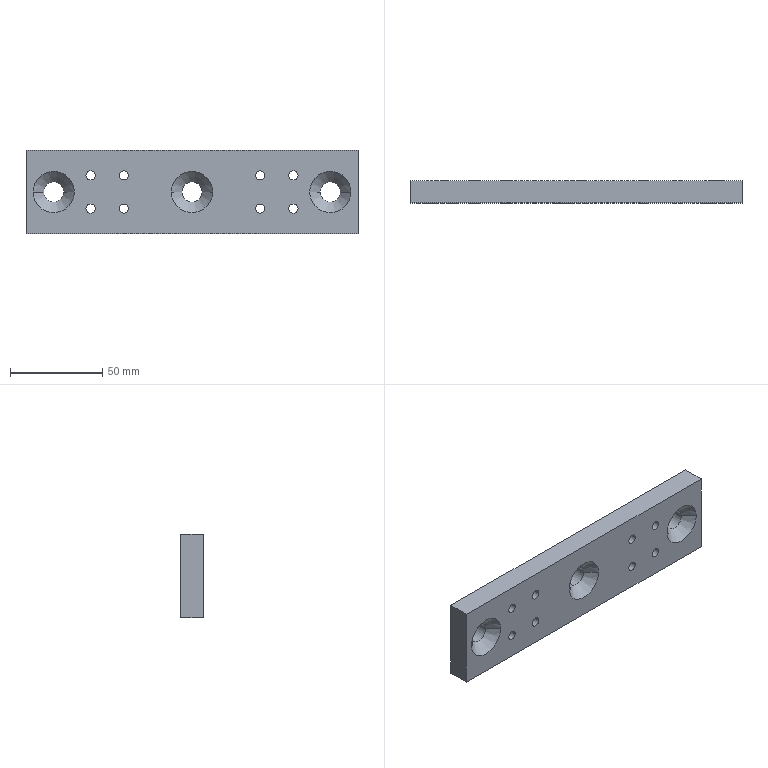Component | SolidWorks | YS01-054ClampingBlockMountingPlate-2 | 1 solid | 34 faces | box 180 x 12 x 45 mm | volume 89628 mm3 | cylinder 22 | cone 6 | plane 6 | commonest cylinder face diameters 5 x16 11 x6
STEP:
#1=COLOUR_RGB('',0.7922,0.8196,0.9333);
#2=FILL_AREA_STYLE_COLOUR('',#1);
#3=FILL_AREA_STYLE('',(#2));
#4=SURFACE_STYLE_FILL_AREA(#3);
#5=SURFACE_SIDE_STYLE('',(#4));
#6=SURFACE_STYLE_USAGE(.BOTH.,#5);
#7=PRESENTATION_STYLE_ASSIGNMENT((#6));
#8=CARTESIAN_POINT('',(-22.091,-12.408,94.425));
#9=VERTEX_POINT('',#8);
#10=CARTESIAN_POINT('',(-22.524,-12.408,94.425));
#11=VERTEX_POINT('',#10);
#12=CARTESIAN_POINT('',(-22.308,-12.408,94.425));
#13=DIRECTION('',(0.,-1.,0.));
#14=DIRECTION('',(-1.,0.,0.));
#15=AXIS2_PLACEMENT_3D('',#12,#13,#14);
#16=CIRCLE('',#15,0.2165);
#17=EDGE_CURVE('',#9,#11,#16,.T.);
#18=ORIENTED_EDGE('',*,*,#17,.F.);
#19=CARTESIAN_POINT('',(-21.867,-12.633,94.425));
#20=VERTEX_POINT('',#19);
#21=CARTESIAN_POINT('',(-21.867,-12.633,94.425));
#22=DIRECTION('',(0.7071,-0.7071,-0.));
#23=VECTOR('',#22,39.37);
#24=LINE('',#21,#23);
#25=EDGE_CURVE('',#9,#20,#24,.T.);
#26=ORIENTED_EDGE('',*,*,#25,.T.);
#27=CARTESIAN_POINT('',(-22.749,-12.633,94.425));
#28=VERTEX_POINT('',#27);
#29=CARTESIAN_POINT('',(-22.308,-12.633,94.425));
#30=DIRECTION('',(0.,-1.,0.));
#31=DIRECTION('',(-1.,0.,0.));
#32=AXIS2_PLACEMENT_3D('',#29,#30,#31);
#33=CIRCLE('',#32,0.4409);
#34=EDGE_CURVE('',#20,#28,#33,.T.);
#35=ORIENTED_EDGE('',*,*,#34,.T.);
#36=CARTESIAN_POINT('',(-22.749,-12.633,94.425));
#37=DIRECTION('',(-0.7071,-0.7071,0.));
#38=VECTOR('',#37,39.37);
#39=LINE('',#36,#38);
#40=EDGE_CURVE('',#11,#28,#39,.T.);
#41=ORIENTED_EDGE('',*,*,#40,.F.);
#42=EDGE_LOOP('',(#18,#26,#35,#41));
#43=FACE_OUTER_BOUND('',#42,.T.);
#44=CARTESIAN_POINT('',(-22.308,-12.633,94.425));
#45=DIRECTION('',(0.,-1.,0.));
#46=DIRECTION('',(-1.,0.,0.));
#47=AXIS2_PLACEMENT_3D('',#44,#45,#46);
#48=CONICAL_SURFACE('',#47,0.4409,0.7854);
#49=ADVANCED_FACE('',(#43),#48,.F.);
#50=CARTESIAN_POINT('',(-22.091,-12.16,94.425));
#51=VERTEX_POINT('',#50);
#52=CARTESIAN_POINT('',(-22.524,-12.16,94.425));
#53=VERTEX_POINT('',#52);
#54=CARTESIAN_POINT('',(-22.308,-12.16,94.425));
#55=DIRECTION('',(0.,-1.,0.));
#56=DIRECTION('',(-1.,0.,0.));
#57=AXIS2_PLACEMENT_3D('',#54,#55,#56);
#58=CIRCLE('',#57,0.2165);
#59=EDGE_CURVE('',#51,#53,#58,.T.);
#60=ORIENTED_EDGE('',*,*,#59,.F.);
#61=CARTESIAN_POINT('',(-22.091,-12.633,94.425));
#62=DIRECTION('',(0.,-1.,0.));
#63=VECTOR('',#62,39.37);
#64=LINE('',#61,#63);
#65=EDGE_CURVE('',#51,#9,#64,.T.);
#66=ORIENTED_EDGE('',*,*,#65,.T.);
#67=ORIENTED_EDGE('',*,*,#17,.T.);
#68=CARTESIAN_POINT('',(-22.524,-12.633,94.425));
#69=DIRECTION('',(0.,-1.,0.));
#70=VECTOR('',#69,39.37);
#71=LINE('',#68,#70);
#72=EDGE_CURVE('',#53,#11,#71,.T.);
#73=ORIENTED_EDGE('',*,*,#72,.F.);
#74=EDGE_LOOP('',(#60,#66,#67,#73));
#75=FACE_OUTER_BOUND('',#74,.T.);
#76=CARTESIAN_POINT('',(-22.308,-12.633,94.425));
#77=DIRECTION('',(0.,-1.,0.));
#78=DIRECTION('',(-1.,0.,0.));
#79=AXIS2_PLACEMENT_3D('',#76,#77,#78);
#80=CYLINDRICAL_SURFACE('',#79,0.2165);
#81=ADVANCED_FACE('',(#75),#80,.F.);
#82=CARTESIAN_POINT('',(-19.138,-12.408,94.425));
#83=VERTEX_POINT('',#82);
#84=CARTESIAN_POINT('',(-19.571,-12.408,94.425));
#85=VERTEX_POINT('',#84);
#86=CARTESIAN_POINT('',(-19.355,-12.408,94.425));
#87=DIRECTION('',(0.,-1.,0.));
#88=DIRECTION('',(-1.,0.,0.));
#89=AXIS2_PLACEMENT_3D('',#86,#87,#88);
#90=CIRCLE('',#89,0.2165);
#91=EDGE_CURVE('',#83,#85,#90,.T.);
#92=ORIENTED_EDGE('',*,*,#91,.F.);
#93=CARTESIAN_POINT('',(-18.914,-12.633,94.425));
#94=VERTEX_POINT('',#93);
#95=CARTESIAN_POINT('',(-18.914,-12.633,94.425));
#96=DIRECTION('',(0.7071,-0.7071,-0.));
#97=VECTOR('',#96,39.37);
#98=LINE('',#95,#97);
#99=EDGE_CURVE('',#83,#94,#98,.T.);
#100=ORIENTED_EDGE('',*,*,#99,.T.);
#101=CARTESIAN_POINT('',(-19.796,-12.633,94.425));
#102=VERTEX_POINT('',#101);
#103=CARTESIAN_POINT('',(-19.355,-12.633,94.425));
#104=DIRECTION('',(0.,-1.,0.));
#105=DIRECTION('',(-1.,0.,0.));
#106=AXIS2_PLACEMENT_3D('',#103,#104,#105);
#107=CIRCLE('',#106,0.4409);
#108=EDGE_CURVE('',#94,#102,#107,.T.);
#109=ORIENTED_EDGE('',*,*,#108,.T.);
#110=CARTESIAN_POINT('',(-19.796,-12.633,94.425));
#111=DIRECTION('',(-0.7071,-0.7071,0.));
#112=VECTOR('',#111,39.37);
#113=LINE('',#110,#112);
#114=EDGE_CURVE('',#85,#102,#113,.T.);
#115=ORIENTED_EDGE('',*,*,#114,.F.);
#116=EDGE_LOOP('',(#92,#100,#109,#115));
#117=FACE_OUTER_BOUND('',#116,.T.);
#118=CARTESIAN_POINT('',(-19.355,-12.633,94.425));
#119=DIRECTION('',(0.,-1.,0.));
#120=DIRECTION('',(-1.,0.,0.));
#121=AXIS2_PLACEMENT_3D('',#118,#119,#120);
#122=CONICAL_SURFACE('',#121,0.4409,0.7854);
#123=ADVANCED_FACE('',(#117),#122,.F.);
#124=CARTESIAN_POINT('',(-19.138,-12.16,94.425));
#125=VERTEX_POINT('',#124);
#126=CARTESIAN_POINT('',(-19.571,-12.16,94.425));
#127=VERTEX_POINT('',#126);
#128=CARTESIAN_POINT('',(-19.355,-12.16,94.425));
#129=DIRECTION('',(0.,-1.,0.));
#130=DIRECTION('',(-1.,0.,0.));
#131=AXIS2_PLACEMENT_3D('',#128,#129,#130);
#132=CIRCLE('',#131,0.2165);
#133=EDGE_CURVE('',#125,#127,#132,.T.);
#134=ORIENTED_EDGE('',*,*,#133,.F.);
#135=CARTESIAN_POINT('',(-19.138,-12.633,94.425));
#136=DIRECTION('',(0.,-1.,0.));
#137=VECTOR('',#136,39.37);
#138=LINE('',#135,#137);
#139=EDGE_CURVE('',#125,#83,#138,.T.);
#140=ORIENTED_EDGE('',*,*,#139,.T.);
#141=ORIENTED_EDGE('',*,*,#91,.T.);
#142=CARTESIAN_POINT('',(-19.571,-12.633,94.425));
#143=DIRECTION('',(0.,-1.,0.));
#144=VECTOR('',#143,39.37);
#145=LINE('',#142,#144);
#146=EDGE_CURVE('',#127,#85,#145,.T.);
#147=ORIENTED_EDGE('',*,*,#146,.F.);
#148=EDGE_LOOP('',(#134,#140,#141,#147));
#149=FACE_OUTER_BOUND('',#148,.T.);
#150=CARTESIAN_POINT('',(-19.355,-12.633,94.425));
#151=DIRECTION('',(0.,-1.,0.));
#152=DIRECTION('',(-1.,0.,0.));
#153=AXIS2_PLACEMENT_3D('',#150,#151,#152);
#154=CYLINDRICAL_SURFACE('',#153,0.2165);
#155=ADVANCED_FACE('',(#149),#154,.F.);
#156=CARTESIAN_POINT('',(-25.044,-12.408,94.425));
#157=VERTEX_POINT('',#156);
#158=CARTESIAN_POINT('',(-25.477,-12.408,94.425));
#159=VERTEX_POINT('',#158);
#160=CARTESIAN_POINT('',(-25.26,-12.408,94.425));
#161=DIRECTION('',(0.,-1.,0.));
#162=DIRECTION('',(-1.,0.,0.));
#163=AXIS2_PLACEMENT_3D('',#160,#161,#162);
#164=CIRCLE('',#163,0.2165);
#165=EDGE_CURVE('',#157,#159,#164,.T.);
#166=ORIENTED_EDGE('',*,*,#165,.F.);
#167=CARTESIAN_POINT('',(-24.819,-12.633,94.425));
#168=VERTEX_POINT('',#167);
#169=CARTESIAN_POINT('',(-24.819,-12.633,94.425));
#170=DIRECTION('',(0.7071,-0.7071,-0.));
#171=VECTOR('',#170,39.37);
#172=LINE('',#169,#171);
#173=EDGE_CURVE('',#157,#168,#172,.T.);
#174=ORIENTED_EDGE('',*,*,#173,.T.);
#175=CARTESIAN_POINT('',(-25.701,-12.633,94.425));
#176=VERTEX_POINT('',#175);
#177=CARTESIAN_POINT('',(-25.26,-12.633,94.425));
#178=DIRECTION('',(0.,-1.,0.));
#179=DIRECTION('',(-1.,0.,0.));
#180=AXIS2_PLACEMENT_3D('',#177,#178,#179);
#181=CIRCLE('',#180,0.4409);
#182=EDGE_CURVE('',#168,#176,#181,.T.);
#183=ORIENTED_EDGE('',*,*,#182,.T.);
#184=CARTESIAN_POINT('',(-25.701,-12.633,94.425));
#185=DIRECTION('',(-0.7071,-0.7071,0.));
#186=VECTOR('',#185,39.37);
#187=LINE('',#184,#186);
#188=EDGE_CURVE('',#159,#176,#187,.T.);
#189=ORIENTED_EDGE('',*,*,#188,.F.);
#190=EDGE_LOOP('',(#166,#174,#183,#189));
#191=FACE_OUTER_BOUND('',#190,.T.);
#192=CARTESIAN_POINT('',(-25.26,-12.633,94.425));
#193=DIRECTION('',(0.,-1.,0.));
#194=DIRECTION('',(-1.,0.,0.));
#195=AXIS2_PLACEMENT_3D('',#192,#193,#194);
#196=CONICAL_SURFACE('',#195,0.4409,0.7854);
#197=ADVANCED_FACE('',(#191),#196,.F.);
#198=CARTESIAN_POINT('',(-25.044,-12.16,94.425));
#199=VERTEX_POINT('',#198);
#200=CARTESIAN_POINT('',(-25.477,-12.16,94.425));
#201=VERTEX_POINT('',#200);
#202=CARTESIAN_POINT('',(-25.26,-12.16,94.425));
#203=DIRECTION('',(0.,-1.,0.));
#204=DIRECTION('',(-1.,0.,0.));
#205=AXIS2_PLACEMENT_3D('',#202,#203,#204);
#206=CIRCLE('',#205,0.2165);
#207=EDGE_CURVE('',#199,#201,#206,.T.);
#208=ORIENTED_EDGE('',*,*,#207,.F.);
#209=CARTESIAN_POINT('',(-25.044,-12.633,94.425));
#210=DIRECTION('',(0.,-1.,0.));
#211=VECTOR('',#210,39.37);
#212=LINE('',#209,#211);
#213=EDGE_CURVE('',#199,#157,#212,.T.);
#214=ORIENTED_EDGE('',*,*,#213,.T.);
#215=ORIENTED_EDGE('',*,*,#165,.T.);
#216=CARTESIAN_POINT('',(-25.477,-12.633,94.425));
#217=DIRECTION('',(0.,-1.,0.));
#218=VECTOR('',#217,39.37);
#219=LINE('',#216,#218);
#220=EDGE_CURVE('',#201,#159,#219,.T.);
#221=ORIENTED_EDGE('',*,*,#220,.F.);
#222=EDGE_LOOP('',(#208,#214,#215,#221));
#223=FACE_OUTER_BOUND('',#222,.T.);
#224=CARTESIAN_POINT('',(-25.26,-12.633,94.425));
#225=DIRECTION('',(0.,-1.,0.));
#226=DIRECTION('',(-1.,0.,0.));
#227=AXIS2_PLACEMENT_3D('',#224,#225,#226);
#228=CYLINDRICAL_SURFACE('',#227,0.2165);
#229=ADVANCED_FACE('',(#223),#228,.F.);
#230=CARTESIAN_POINT('',(-23.863,-12.16,94.071));
#231=VERTEX_POINT('',#230);
#232=CARTESIAN_POINT('',(-23.666,-12.16,94.071));
#233=VERTEX_POINT('',#232);
#234=CARTESIAN_POINT('',(-23.764,-12.16,94.071));
#235=DIRECTION('',(-0.,1.,0.));
#236=DIRECTION('',(1.,0.,0.));
#237=AXIS2_PLACEMENT_3D('',#234,#235,#236);
#238=CIRCLE('',#237,0.09843);
#239=EDGE_CURVE('',#231,#233,#238,.T.);
#240=ORIENTED_EDGE('',*,*,#239,.T.);
#241=CARTESIAN_POINT('',(-23.666,-12.633,94.071));
#242=VERTEX_POINT('',#241);
#243=CARTESIAN_POINT('',(-23.666,-12.633,94.071));
#244=DIRECTION('',(0.,-1.,0.));
#245=VECTOR('',#244,39.37);
#246=LINE('',#243,#245);
#247=EDGE_CURVE('',#233,#242,#246,.T.);
#248=ORIENTED_EDGE('',*,*,#247,.T.);
#249=CARTESIAN_POINT('',(-23.863,-12.633,94.071));
#250=VERTEX_POINT('',#249);
#251=CARTESIAN_POINT('',(-23.764,-12.633,94.071));
#252=DIRECTION('',(0.,-1.,0.));
#253=DIRECTION('',(-1.,0.,0.));
#254=AXIS2_PLACEMENT_3D('',#251,#252,#253);
#255=CIRCLE('',#254,0.09843);
#256=EDGE_CURVE('',#242,#250,#255,.T.);
#257=ORIENTED_EDGE('',*,*,#256,.T.);
#258=CARTESIAN_POINT('',(-23.863,-12.633,94.071));
#259=DIRECTION('',(0.,-1.,0.));
#260=VECTOR('',#259,39.37);
#261=LINE('',#258,#260);
#262=EDGE_CURVE('',#231,#250,#261,.T.);
#263=ORIENTED_EDGE('',*,*,#262,.F.);
#264=EDGE_LOOP('',(#240,#248,#257,#263));
#265=FACE_OUTER_BOUND('',#264,.T.);
#266=CARTESIAN_POINT('',(-23.764,-12.633,94.071));
#267=DIRECTION('',(0.,-1.,0.));
#268=DIRECTION('',(-1.,0.,0.));
#269=AXIS2_PLACEMENT_3D('',#266,#267,#268);
#270=CYLINDRICAL_SURFACE('',#269,0.09843);
#271=ADVANCED_FACE('',(#265),#270,.F.);
#272=CARTESIAN_POINT('',(-20.949,-12.16,94.071));
#273=VERTEX_POINT('',#272);
#274=CARTESIAN_POINT('',(-20.752,-12.16,94.071));
#275=VERTEX_POINT('',#274);
#276=CARTESIAN_POINT('',(-20.851,-12.16,94.071));
#277=DIRECTION('',(-0.,1.,0.));
#278=DIRECTION('',(1.,0.,0.));
#279=AXIS2_PLACEMENT_3D('',#276,#277,#278);
#280=CIRCLE('',#279,0.09843);
#281=EDGE_CURVE('',#273,#275,#280,.T.);
#282=ORIENTED_EDGE('',*,*,#281,.T.);
#283=CARTESIAN_POINT('',(-20.752,-12.633,94.071));
#284=VERTEX_POINT('',#283);
#285=CARTESIAN_POINT('',(-20.752,-12.633,94.071));
#286=DIRECTION('',(0.,-1.,0.));
#287=VECTOR('',#286,39.37);
#288=LINE('',#285,#287);
#289=EDGE_CURVE('',#275,#284,#288,.T.);
#290=ORIENTED_EDGE('',*,*,#289,.T.);
#291=CARTESIAN_POINT('',(-20.949,-12.633,94.071));
#292=VERTEX_POINT('',#291);
#293=CARTESIAN_POINT('',(-20.851,-12.633,94.071));
#294=DIRECTION('',(0.,-1.,0.));
#295=DIRECTION('',(-1.,0.,0.));
#296=AXIS2_PLACEMENT_3D('',#293,#294,#295);
#297=CIRCLE('',#296,0.09843);
#298=EDGE_CURVE('',#284,#292,#297,.T.);
#299=ORIENTED_EDGE('',*,*,#298,.T.);
#300=CARTESIAN_POINT('',(-20.949,-12.633,94.071));
#301=DIRECTION('',(0.,-1.,0.));
#302=VECTOR('',#301,39.37);
#303=LINE('',#300,#302);
#304=EDGE_CURVE('',#273,#292,#303,.T.);
#305=ORIENTED_EDGE('',*,*,#304,.F.);
#306=EDGE_LOOP('',(#282,#290,#299,#305));
#307=FACE_OUTER_BOUND('',#306,.T.);
#308=CARTESIAN_POINT('',(-20.851,-12.633,94.071));
#309=DIRECTION('',(0.,-1.,0.));
#310=DIRECTION('',(-1.,0.,0.));
#311=AXIS2_PLACEMENT_3D('',#308,#309,#310);
#312=CYLINDRICAL_SURFACE('',#311,0.09843);
#313=ADVANCED_FACE('',(#307),#312,.F.);
#314=CARTESIAN_POINT('',(-23.863,-12.16,94.78));
#315=VERTEX_POINT('',#314);
#316=CARTESIAN_POINT('',(-23.666,-12.16,94.78));
#317=VERTEX_POINT('',#316);
#318=CARTESIAN_POINT('',(-23.764,-12.16,94.78));
#319=DIRECTION('',(-0.,1.,0.));
#320=DIRECTION('',(1.,0.,0.));
#321=AXIS2_PLACEMENT_3D('',#318,#319,#320);
#322=CIRCLE('',#321,0.09843);
#323=EDGE_CURVE('',#315,#317,#322,.T.);
#324=ORIENTED_EDGE('',*,*,#323,.T.);
#325=CARTESIAN_POINT('',(-23.666,-12.633,94.78));
#326=VERTEX_POINT('',#325);
#327=CARTESIAN_POINT('',(-23.666,-12.633,94.78));
#328=DIRECTION('',(0.,-1.,0.));
#329=VECTOR('',#328,39.37);
#330=LINE('',#327,#329);
#331=EDGE_CURVE('',#317,#326,#330,.T.);
#332=ORIENTED_EDGE('',*,*,#331,.T.);
#333=CARTESIAN_POINT('',(-23.863,-12.633,94.78));
#334=VERTEX_POINT('',#333);
#335=CARTESIAN_POINT('',(-23.764,-12.633,94.78));
#336=DIRECTION('',(0.,-1.,0.));
#337=DIRECTION('',(-1.,0.,0.));
#338=AXIS2_PLACEMENT_3D('',#335,#336,#337);
#339=CIRCLE('',#338,0.09843);
#340=EDGE_CURVE('',#326,#334,#339,.T.);
#341=ORIENTED_EDGE('',*,*,#340,.T.);
#342=CARTESIAN_POINT('',(-23.863,-12.633,94.78));
#343=DIRECTION('',(0.,-1.,0.));
#344=VECTOR('',#343,39.37);
#345=LINE('',#342,#344);
#346=EDGE_CURVE('',#315,#334,#345,.T.);
#347=ORIENTED_EDGE('',*,*,#346,.F.);
#348=EDGE_LOOP('',(#324,#332,#341,#347));
#349=FACE_OUTER_BOUND('',#348,.T.);
#350=CARTESIAN_POINT('',(-23.764,-12.633,94.78));
#351=DIRECTION('',(0.,-1.,0.));
#352=DIRECTION('',(-1.,0.,0.));
#353=AXIS2_PLACEMENT_3D('',#350,#351,#352);
#354=CYLINDRICAL_SURFACE('',#353,0.09843);
#355=ADVANCED_FACE('',(#349),#354,.F.);
#356=CARTESIAN_POINT('',(-20.949,-12.16,94.78));
#357=VERTEX_POINT('',#356);
#358=CARTESIAN_POINT('',(-20.752,-12.16,94.78));
#359=VERTEX_POINT('',#358);
#360=CARTESIAN_POINT('',(-20.851,-12.16,94.78));
#361=DIRECTION('',(-0.,1.,0.));
#362=DIRECTION('',(1.,0.,0.));
#363=AXIS2_PLACEMENT_3D('',#360,#361,#362);
#364=CIRCLE('',#363,0.09843);
#365=EDGE_CURVE('',#357,#359,#364,.T.);
#366=ORIENTED_EDGE('',*,*,#365,.T.);
#367=CARTESIAN_POINT('',(-20.752,-12.633,94.78));
#368=VERTEX_POINT('',#367);
#369=CARTESIAN_POINT('',(-20.752,-12.633,94.78));
#370=DIRECTION('',(0.,-1.,0.));
#371=VECTOR('',#370,39.37);
#372=LINE('',#369,#371);
#373=EDGE_CURVE('',#359,#368,#372,.T.);
#374=ORIENTED_EDGE('',*,*,#373,.T.);
#375=CARTESIAN_POINT('',(-20.949,-12.633,94.78));
#376=VERTEX_POINT('',#375);
#377=CARTESIAN_POINT('',(-20.851,-12.633,94.78));
#378=DIRECTION('',(0.,-1.,0.));
#379=DIRECTION('',(-1.,0.,0.));
#380=AXIS2_PLACEMENT_3D('',#377,#378,#379);
#381=CIRCLE('',#380,0.09843);
#382=EDGE_CURVE('',#368,#376,#381,.T.);
#383=ORIENTED_EDGE('',*,*,#382,.T.);
#384=CARTESIAN_POINT('',(-20.949,-12.633,94.78));
#385=DIRECTION('',(0.,-1.,0.));
#386=VECTOR('',#385,39.37);
#387=LINE('',#384,#386);
#388=EDGE_CURVE('',#357,#376,#387,.T.);
#389=ORIENTED_EDGE('',*,*,#388,.F.);
#390=EDGE_LOOP('',(#366,#374,#383,#389));
#391=FACE_OUTER_BOUND('',#390,.T.);
#392=CARTESIAN_POINT('',(-20.851,-12.633,94.78));
#393=DIRECTION('',(0.,-1.,0.));
#394=DIRECTION('',(-1.,0.,0.));
#395=AXIS2_PLACEMENT_3D('',#392,#393,#394);
#396=CYLINDRICAL_SURFACE('',#395,0.09843);
#397=ADVANCED_FACE('',(#391),#396,.F.);
#398=CARTESIAN_POINT('',(-24.571,-12.16,94.78));
#399=VERTEX_POINT('',#398);
#400=CARTESIAN_POINT('',(-24.374,-12.16,94.78));
#401=VERTEX_POINT('',#400);
#402=CARTESIAN_POINT('',(-24.473,-12.16,94.78));
#403=DIRECTION('',(-0.,1.,0.));
#404=DIRECTION('',(1.,0.,0.));
#405=AXIS2_PLACEMENT_3D('',#402,#403,#404);
#406=CIRCLE('',#405,0.09843);
#407=EDGE_CURVE('',#399,#401,#406,.T.);
#408=ORIENTED_EDGE('',*,*,#407,.T.);
#409=CARTESIAN_POINT('',(-24.374,-12.633,94.78));
#410=VERTEX_POINT('',#409);
#411=CARTESIAN_POINT('',(-24.374,-12.633,94.78));
#412=DIRECTION('',(0.,-1.,0.));
#413=VECTOR('',#412,39.37);
#414=LINE('',#411,#413);
#415=EDGE_CURVE('',#401,#410,#414,.T.);
#416=ORIENTED_EDGE('',*,*,#415,.T.);
#417=CARTESIAN_POINT('',(-24.571,-12.633,94.78));
#418=VERTEX_POINT('',#417);
#419=CARTESIAN_POINT('',(-24.473,-12.633,94.78));
#420=DIRECTION('',(0.,-1.,0.));
#421=DIRECTION('',(-1.,0.,0.));
#422=AXIS2_PLACEMENT_3D('',#419,#420,#421);
#423=CIRCLE('',#422,0.09843);
#424=EDGE_CURVE('',#410,#418,#423,.T.);
#425=ORIENTED_EDGE('',*,*,#424,.T.);
#426=CARTESIAN_POINT('',(-24.571,-12.633,94.78));
#427=DIRECTION('',(0.,-1.,0.));
#428=VECTOR('',#427,39.37);
#429=LINE('',#426,#428);
#430=EDGE_CURVE('',#399,#418,#429,.T.);
#431=ORIENTED_EDGE('',*,*,#430,.F.);
#432=EDGE_LOOP('',(#408,#416,#425,#431));
#433=FACE_OUTER_BOUND('',#432,.T.);
#434=CARTESIAN_POINT('',(-24.473,-12.633,94.78));
#435=DIRECTION('',(0.,-1.,0.));
#436=DIRECTION('',(-1.,0.,0.));
#437=AXIS2_PLACEMENT_3D('',#434,#435,#436);
#438=CYLINDRICAL_SURFACE('',#437,0.09843);
#439=ADVANCED_FACE('',(#433),#438,.F.);
#440=CARTESIAN_POINT('',(-24.571,-12.16,94.071));
#441=VERTEX_POINT('',#440);
#442=CARTESIAN_POINT('',(-24.374,-12.16,94.071));
#443=VERTEX_POINT('',#442);
#444=CARTESIAN_POINT('',(-24.473,-12.16,94.071));
#445=DIRECTION('',(-0.,1.,0.));
#446=DIRECTION('',(1.,0.,0.));
#447=AXIS2_PLACEMENT_3D('',#444,#445,#446);
#448=CIRCLE('',#447,0.09843);
#449=EDGE_CURVE('',#441,#443,#448,.T.);
#450=ORIENTED_EDGE('',*,*,#449,.T.);
#451=CARTESIAN_POINT('',(-24.374,-12.633,94.071));
#452=VERTEX_POINT('',#451);
#453=CARTESIAN_POINT('',(-24.374,-12.633,94.071));
#454=DIRECTION('',(0.,-1.,0.));
#455=VECTOR('',#454,39.37);
#456=LINE('',#453,#455);
#457=EDGE_CURVE('',#443,#452,#456,.T.);
#458=ORIENTED_EDGE('',*,*,#457,.T.);
#459=CARTESIAN_POINT('',(-24.571,-12.633,94.071));
#460=VERTEX_POINT('',#459);
#461=CARTESIAN_POINT('',(-24.473,-12.633,94.071));
#462=DIRECTION('',(0.,-1.,0.));
#463=DIRECTION('',(-1.,0.,0.));
#464=AXIS2_PLACEMENT_3D('',#461,#462,#463);
#465=CIRCLE('',#464,0.09843);
#466=EDGE_CURVE('',#452,#460,#465,.T.);
#467=ORIENTED_EDGE('',*,*,#466,.T.);
#468=CARTESIAN_POINT('',(-24.571,-12.633,94.071));
#469=DIRECTION('',(0.,-1.,0.));
#470=VECTOR('',#469,39.37);
#471=LINE('',#468,#470);
#472=EDGE_CURVE('',#441,#460,#471,.T.);
#473=ORIENTED_EDGE('',*,*,#472,.F.);
#474=EDGE_LOOP('',(#450,#458,#467,#473));
#475=FACE_OUTER_BOUND('',#474,.T.);
#476=CARTESIAN_POINT('',(-24.473,-12.633,94.071));
#477=DIRECTION('',(0.,-1.,0.));
#478=DIRECTION('',(-1.,0.,0.));
#479=AXIS2_PLACEMENT_3D('',#476,#477,#478);
#480=CYLINDRICAL_SURFACE('',#479,0.09843);
#481=ADVANCED_FACE('',(#475),#480,.F.);
#482=CARTESIAN_POINT('',(-20.241,-12.16,94.78));
#483=VERTEX_POINT('',#482);
#484=CARTESIAN_POINT('',(-20.044,-12.16,94.78));
#485=VERTEX_POINT('',#484);
#486=CARTESIAN_POINT('',(-20.142,-12.16,94.78));
#487=DIRECTION('',(-0.,1.,0.));
#488=DIRECTION('',(1.,0.,0.));
#489=AXIS2_PLACEMENT_3D('',#486,#487,#488);
#490=CIRCLE('',#489,0.09843);
#491=EDGE_CURVE('',#483,#485,#490,.T.);
#492=ORIENTED_EDGE('',*,*,#491,.T.);
#493=CARTESIAN_POINT('',(-20.044,-12.633,94.78));
#494=VERTEX_POINT('',#493);
#495=CARTESIAN_POINT('',(-20.044,-12.633,94.78));
#496=DIRECTION('',(0.,-1.,0.));
#497=VECTOR('',#496,39.37);
#498=LINE('',#495,#497);
#499=EDGE_CURVE('',#485,#494,#498,.T.);
#500=ORIENTED_EDGE('',*,*,#499,.T.);
#501=CARTESIAN_POINT('',(-20.241,-12.633,94.78));
#502=VERTEX_POINT('',#501);
#503=CARTESIAN_POINT('',(-20.142,-12.633,94.78));
#504=DIRECTION('',(0.,-1.,0.));
#505=DIRECTION('',(-1.,0.,0.));
#506=AXIS2_PLACEMENT_3D('',#503,#504,#505);
#507=CIRCLE('',#506,0.09843);
#508=EDGE_CURVE('',#494,#502,#507,.T.);
#509=ORIENTED_EDGE('',*,*,#508,.T.);
#510=CARTESIAN_POINT('',(-20.241,-12.633,94.78));
#511=DIRECTION('',(0.,-1.,0.));
#512=VECTOR('',#511,39.37);
#513=LINE('',#510,#512);
#514=EDGE_CURVE('',#483,#502,#513,.T.);
#515=ORIENTED_EDGE('',*,*,#514,.F.);
#516=EDGE_LOOP('',(#492,#500,#509,#515));
#517=FACE_OUTER_BOUND('',#516,.T.);
#518=CARTESIAN_POINT('',(-20.142,-12.633,94.78));
#519=DIRECTION('',(0.,-1.,0.));
#520=DIRECTION('',(-1.,0.,0.));
#521=AXIS2_PLACEMENT_3D('',#518,#519,#520);
#522=CYLINDRICAL_SURFACE('',#521,0.09843);
#523=ADVANCED_FACE('',(#517),#522,.F.);
#524=CARTESIAN_POINT('',(-20.241,-12.16,94.071));
#525=VERTEX_POINT('',#524);
#526=CARTESIAN_POINT('',(-20.044,-12.16,94.071));
#527=VERTEX_POINT('',#526);
#528=CARTESIAN_POINT('',(-20.142,-12.16,94.071));
#529=DIRECTION('',(-0.,1.,0.));
#530=DIRECTION('',(1.,0.,0.));
#531=AXIS2_PLACEMENT_3D('',#528,#529,#530);
#532=CIRCLE('',#531,0.09843);
#533=EDGE_CURVE('',#525,#527,#532,.T.);
#534=ORIENTED_EDGE('',*,*,#533,.T.);
#535=CARTESIAN_POINT('',(-20.044,-12.633,94.071));
#536=VERTEX_POINT('',#535);
#537=CARTESIAN_POINT('',(-20.044,-12.633,94.071));
#538=DIRECTION('',(0.,-1.,0.));
#539=VECTOR('',#538,39.37);
#540=LINE('',#537,#539);
#541=EDGE_CURVE('',#527,#536,#540,.T.);
#542=ORIENTED_EDGE('',*,*,#541,.T.);
#543=CARTESIAN_POINT('',(-20.241,-12.633,94.071));
#544=VERTEX_POINT('',#543);
#545=CARTESIAN_POINT('',(-20.142,-12.633,94.071));
#546=DIRECTION('',(0.,-1.,0.));
#547=DIRECTION('',(-1.,0.,0.));
#548=AXIS2_PLACEMENT_3D('',#545,#546,#547);
#549=CIRCLE('',#548,0.09843);
#550=EDGE_CURVE('',#536,#544,#549,.T.);
#551=ORIENTED_EDGE('',*,*,#550,.T.);
#552=CARTESIAN_POINT('',(-20.241,-12.633,94.071));
#553=DIRECTION('',(0.,-1.,0.));
#554=VECTOR('',#553,39.37);
#555=LINE('',#552,#554);
#556=EDGE_CURVE('',#525,#544,#555,.T.);
#557=ORIENTED_EDGE('',*,*,#556,.F.);
#558=EDGE_LOOP('',(#534,#542,#551,#557));
#559=FACE_OUTER_BOUND('',#558,.T.);
#560=CARTESIAN_POINT('',(-20.142,-12.633,94.071));
#561=DIRECTION('',(0.,-1.,0.));
#562=DIRECTION('',(-1.,0.,0.));
#563=AXIS2_PLACEMENT_3D('',#560,#561,#562);
#564=CYLINDRICAL_SURFACE('',#563,0.09843);
#565=ADVANCED_FACE('',(#559),#564,.F.);
#566=CARTESIAN_POINT('',(-22.308,-12.633,94.425));
#567=DIRECTION('',(0.,-1.,0.));
#568=DIRECTION('',(-1.,0.,0.));
#569=AXIS2_PLACEMENT_3D('',#566,#567,#568);
#570=CIRCLE('',#569,0.4409);
#571=EDGE_CURVE('',#28,#20,#570,.T.);
#572=ORIENTED_EDGE('',*,*,#571,.F.);
#573=ORIENTED_EDGE('',*,*,#34,.F.);
#574=EDGE_LOOP('',(#572,#573));
#575=FACE_BOUND('',#574,.T.);
#576=CARTESIAN_POINT('',(-19.355,-12.633,94.425));
#577=DIRECTION('',(0.,-1.,0.));
#578=DIRECTION('',(-1.,0.,0.));
#579=AXIS2_PLACEMENT_3D('',#576,#577,#578);
#580=CIRCLE('',#579,0.4409);
#581=EDGE_CURVE('',#102,#94,#580,.T.);
#582=ORIENTED_EDGE('',*,*,#581,.F.);
#583=ORIENTED_EDGE('',*,*,#108,.F.);
#584=EDGE_LOOP('',(#582,#583));
#585=FACE_BOUND('',#584,.T.);
#586=CARTESIAN_POINT('',(-25.26,-12.633,94.425));
#587=DIRECTION('',(0.,-1.,0.));
#588=DIRECTION('',(-1.,0.,0.));
#589=AXIS2_PLACEMENT_3D('',#586,#587,#588);
#590=CIRCLE('',#589,0.4409);
#591=EDGE_CURVE('',#176,#168,#590,.T.);
#592=ORIENTED_EDGE('',*,*,#591,.F.);
#593=ORIENTED_EDGE('',*,*,#182,.F.);
#594=EDGE_LOOP('',(#592,#593));
#595=FACE_BOUND('',#594,.T.);
#596=CARTESIAN_POINT('',(-20.851,-12.633,94.071));
#597=DIRECTION('',(0.,-1.,0.));
#598=DIRECTION('',(-1.,0.,0.));
#599=AXIS2_PLACEMENT_3D('',#596,#597,#598);
#600=CIRCLE('',#599,0.09843);
#601=EDGE_CURVE('',#292,#284,#600,.T.);
#602=ORIENTED_EDGE('',*,*,#601,.F.);
#603=ORIENTED_EDGE('',*,*,#298,.F.);
#604=EDGE_LOOP('',(#602,#603));
#605=FACE_BOUND('',#604,.T.);
#606=CARTESIAN_POINT('',(-23.764,-12.633,94.78));
#607=DIRECTION('',(0.,-1.,0.));
#608=DIRECTION('',(-1.,0.,0.));
#609=AXIS2_PLACEMENT_3D('',#606,#607,#608);
#610=CIRCLE('',#609,0.09843);
#611=EDGE_CURVE('',#334,#326,#610,.T.);
#612=ORIENTED_EDGE('',*,*,#611,.F.);
#613=ORIENTED_EDGE('',*,*,#340,.F.);
#614=EDGE_LOOP('',(#612,#613));
#615=FACE_BOUND('',#614,.T.);
#616=CARTESIAN_POINT('',(-20.851,-12.633,94.78));
#617=DIRECTION('',(0.,-1.,0.));
#618=DIRECTION('',(-1.,0.,0.));
#619=AXIS2_PLACEMENT_3D('',#616,#617,#618);
#620=CIRCLE('',#619,0.09843);
#621=EDGE_CURVE('',#376,#368,#620,.T.);
#622=ORIENTED_EDGE('',*,*,#621,.F.);
#623=ORIENTED_EDGE('',*,*,#382,.F.);
#624=EDGE_LOOP('',(#622,#623));
#625=FACE_BOUND('',#624,.T.);
#626=CARTESIAN_POINT('',(-24.473,-12.633,94.78));
#627=DIRECTION('',(0.,-1.,0.));
#628=DIRECTION('',(-1.,0.,0.));
#629=AXIS2_PLACEMENT_3D('',#626,#627,#628);
#630=CIRCLE('',#629,0.09843);
#631=EDGE_CURVE('',#418,#410,#630,.T.);
#632=ORIENTED_EDGE('',*,*,#631,.F.);
#633=ORIENTED_EDGE('',*,*,#424,.F.);
#634=EDGE_LOOP('',(#632,#633));
#635=FACE_BOUND('',#634,.T.);
#636=CARTESIAN_POINT('',(-24.473,-12.633,94.071));
#637=DIRECTION('',(0.,-1.,0.));
#638=DIRECTION('',(-1.,0.,0.));
#639=AXIS2_PLACEMENT_3D('',#636,#637,#638);
#640=CIRCLE('',#639,0.09843);
#641=EDGE_CURVE('',#460,#452,#640,.T.);
#642=ORIENTED_EDGE('',*,*,#641,.F.);
#643=ORIENTED_EDGE('',*,*,#466,.F.);
#644=EDGE_LOOP('',(#642,#643));
#645=FACE_BOUND('',#644,.T.);
#646=CARTESIAN_POINT('',(-20.142,-12.633,94.78));
#647=DIRECTION('',(0.,-1.,0.));
#648=DIRECTION('',(-1.,0.,0.));
#649=AXIS2_PLACEMENT_3D('',#646,#647,#648);
#650=CIRCLE('',#649,0.09843);
#651=EDGE_CURVE('',#502,#494,#650,.T.);
#652=ORIENTED_EDGE('',*,*,#651,.F.);
#653=ORIENTED_EDGE('',*,*,#508,.F.);
#654=EDGE_LOOP('',(#652,#653));
#655=FACE_BOUND('',#654,.T.);
#656=CARTESIAN_POINT('',(-20.142,-12.633,94.071));
#657=DIRECTION('',(0.,-1.,0.));
#658=DIRECTION('',(-1.,0.,0.));
#659=AXIS2_PLACEMENT_3D('',#656,#657,#658);
#660=CIRCLE('',#659,0.09843);
#661=EDGE_CURVE('',#544,#536,#660,.T.);
#662=ORIENTED_EDGE('',*,*,#661,.F.);
#663=ORIENTED_EDGE('',*,*,#550,.F.);
#664=EDGE_LOOP('',(#662,#663));
#665=FACE_BOUND('',#664,.T.);
#666=CARTESIAN_POINT('',(-25.851,-12.633,93.539));
#667=VERTEX_POINT('',#666);
#668=CARTESIAN_POINT('',(-25.851,-12.633,95.311));
#669=VERTEX_POINT('',#668);
#670=CARTESIAN_POINT('',(-25.851,-12.633,93.539));
#671=DIRECTION('',(0.,0.,1.));
#672=VECTOR('',#671,39.37);
#673=LINE('',#670,#672);
#674=EDGE_CURVE('',#667,#669,#673,.T.);
#675=ORIENTED_EDGE('',*,*,#674,.F.);
#676=CARTESIAN_POINT('',(-18.764,-12.633,93.539));
#677=VERTEX_POINT('',#676);
#678=CARTESIAN_POINT('',(-25.851,-12.633,93.539));
#679=DIRECTION('',(-1.,-0.,0.));
#680=VECTOR('',#679,39.37);
#681=LINE('',#678,#680);
#682=EDGE_CURVE('',#677,#667,#681,.T.);
#683=ORIENTED_EDGE('',*,*,#682,.F.);
#684=CARTESIAN_POINT('',(-18.764,-12.633,95.311));
#685=VERTEX_POINT('',#684);
#686=CARTESIAN_POINT('',(-18.764,-12.633,93.539));
#687=DIRECTION('',(-0.,-0.,-1.));
#688=VECTOR('',#687,39.37);
#689=LINE('',#686,#688);
#690=EDGE_CURVE('',#685,#677,#689,.T.);
#691=ORIENTED_EDGE('',*,*,#690,.F.);
#692=CARTESIAN_POINT('',(-25.851,-12.633,95.311));
#693=DIRECTION('',(1.,0.,0.));
#694=VECTOR('',#693,39.37);
#695=LINE('',#692,#694);
#696=EDGE_CURVE('',#669,#685,#695,.T.);
#697=ORIENTED_EDGE('',*,*,#696,.F.);
#698=EDGE_LOOP('',(#675,#683,#691,#697));
#699=FACE_OUTER_BOUND('',#698,.T.);
#700=CARTESIAN_POINT('',(-23.764,-12.633,94.071));
#701=DIRECTION('',(0.,-1.,0.));
#702=DIRECTION('',(-1.,0.,0.));
#703=AXIS2_PLACEMENT_3D('',#700,#701,#702);
#704=CIRCLE('',#703,0.09843);
#705=EDGE_CURVE('',#250,#242,#704,.T.);
#706=ORIENTED_EDGE('',*,*,#705,.F.);
#707=ORIENTED_EDGE('',*,*,#256,.F.);
#708=EDGE_LOOP('',(#706,#707));
#709=FACE_BOUND('',#708,.T.);
#710=CARTESIAN_POINT('',(-23.193,-12.633,92.28));
#711=DIRECTION('',(-0.,1.,0.));
#712=DIRECTION('',(1.,0.,0.));
#713=AXIS2_PLACEMENT_3D('',#710,#711,#712);
#714=PLANE('',#713);
#715=ADVANCED_FACE('',(#575,#585,#595,#605,#615,#625,#635,#645,#655,#665,#699,#709),#714,.F.);
#716=ORIENTED_EDGE('',*,*,#674,.T.);
#717=CARTESIAN_POINT('',(-25.851,-12.16,95.311));
#718=VERTEX_POINT('',#717);
#719=CARTESIAN_POINT('',(-25.851,-12.16,95.311));
#720=DIRECTION('',(0.,-1.,0.));
#721=VECTOR('',#720,39.37);
#722=LINE('',#719,#721);
#723=EDGE_CURVE('',#718,#669,#722,.T.);
#724=ORIENTED_EDGE('',*,*,#723,.F.);
#725=CARTESIAN_POINT('',(-25.851,-12.16,93.539));
#726=VERTEX_POINT('',#725);
#727=CARTESIAN_POINT('',(-25.851,-12.16,93.539));
#728=DIRECTION('',(0.,0.,1.));
#729=VECTOR('',#728,39.37);
#730=LINE('',#727,#729);
#731=EDGE_CURVE('',#726,#718,#730,.T.);
#732=ORIENTED_EDGE('',*,*,#731,.F.);
#733=CARTESIAN_POINT('',(-25.851,-12.16,93.539));
#734=DIRECTION('',(0.,-1.,0.));
#735=VECTOR('',#734,39.37);
#736=LINE('',#733,#735);
#737=EDGE_CURVE('',#726,#667,#736,.T.);
#738=ORIENTED_EDGE('',*,*,#737,.T.);
#739=EDGE_LOOP('',(#716,#724,#732,#738));
#740=FACE_OUTER_BOUND('',#739,.T.);
#741=CARTESIAN_POINT('',(-25.851,-12.16,93.539));
#742=DIRECTION('',(1.,0.,0.));
#743=DIRECTION('',(0.,-1.,0.));
#744=AXIS2_PLACEMENT_3D('',#741,#742,#743);
#745=PLANE('',#744);
#746=ADVANCED_FACE('',(#740),#745,.F.);
#747=ORIENTED_EDGE('',*,*,#696,.T.);
#748=CARTESIAN_POINT('',(-18.764,-12.16,95.311));
#749=VERTEX_POINT('',#748);
#750=CARTESIAN_POINT('',(-18.764,-12.16,95.311));
#751=DIRECTION('',(0.,-1.,0.));
#752=VECTOR('',#751,39.37);
#753=LINE('',#750,#752);
#754=EDGE_CURVE('',#749,#685,#753,.T.);
#755=ORIENTED_EDGE('',*,*,#754,.F.);
#756=CARTESIAN_POINT('',(-25.851,-12.16,95.311));
#757=DIRECTION('',(1.,0.,0.));
#758=VECTOR('',#757,39.37);
#759=LINE('',#756,#758);
#760=EDGE_CURVE('',#718,#749,#759,.T.);
#761=ORIENTED_EDGE('',*,*,#760,.F.);
#762=ORIENTED_EDGE('',*,*,#723,.T.);
#763=EDGE_LOOP('',(#747,#755,#761,#762));
#764=FACE_OUTER_BOUND('',#763,.T.);
#765=CARTESIAN_POINT('',(-25.851,-12.16,95.311));
#766=DIRECTION('',(0.,0.,-1.));
#767=DIRECTION('',(-0.,1.,0.));
#768=AXIS2_PLACEMENT_3D('',#765,#766,#767);
#769=PLANE('',#768);
#770=ADVANCED_FACE('',(#764),#769,.F.);
#771=ORIENTED_EDGE('',*,*,#690,.T.);
#772=CARTESIAN_POINT('',(-18.764,-12.16,93.539));
#773=VERTEX_POINT('',#772);
#774=CARTESIAN_POINT('',(-18.764,-12.16,93.539));
#775=DIRECTION('',(0.,-1.,0.));
#776=VECTOR('',#775,39.37);
#777=LINE('',#774,#776);
#778=EDGE_CURVE('',#773,#677,#777,.T.);
#779=ORIENTED_EDGE('',*,*,#778,.F.);
#780=CARTESIAN_POINT('',(-18.764,-12.16,93.539));
#781=DIRECTION('',(-0.,-0.,-1.));
#782=VECTOR('',#781,39.37);
#783=LINE('',#780,#782);
#784=EDGE_CURVE('',#749,#773,#783,.T.);
#785=ORIENTED_EDGE('',*,*,#784,.F.);
#786=ORIENTED_EDGE('',*,*,#754,.T.);
#787=EDGE_LOOP('',(#771,#779,#785,#786));
#788=FACE_OUTER_BOUND('',#787,.T.);
#789=CARTESIAN_POINT('',(-18.764,-12.16,93.539));
#790=DIRECTION('',(-1.,-0.,0.));
#791=DIRECTION('',(0.,0.,1.));
#792=AXIS2_PLACEMENT_3D('',#789,#790,#791);
#793=PLANE('',#792);
#794=ADVANCED_FACE('',(#788),#793,.F.);
#795=ORIENTED_EDGE('',*,*,#682,.T.);
#796=ORIENTED_EDGE('',*,*,#737,.F.);
#797=CARTESIAN_POINT('',(-25.851,-12.16,93.539));
#798=DIRECTION('',(-1.,-0.,0.));
#799=VECTOR('',#798,39.37);
#800=LINE('',#797,#799);
#801=EDGE_CURVE('',#773,#726,#800,.T.);
#802=ORIENTED_EDGE('',*,*,#801,.F.);
#803=ORIENTED_EDGE('',*,*,#778,.T.);
#804=EDGE_LOOP('',(#795,#796,#802,#803));
#805=FACE_OUTER_BOUND('',#804,.T.);
#806=CARTESIAN_POINT('',(-25.851,-12.16,93.539));
#807=DIRECTION('',(0.,0.,1.));
#808=DIRECTION('',(0.,-1.,0.));
#809=AXIS2_PLACEMENT_3D('',#806,#807,#808);
#810=PLANE('',#809);
#811=ADVANCED_FACE('',(#805),#810,.F.);
#812=CARTESIAN_POINT('',(-22.308,-12.16,94.425));
#813=DIRECTION('',(0.,-1.,0.));
#814=DIRECTION('',(-1.,0.,0.));
#815=AXIS2_PLACEMENT_3D('',#812,#813,#814);
#816=CIRCLE('',#815,0.2165);
#817=EDGE_CURVE('',#53,#51,#816,.T.);
#818=ORIENTED_EDGE('',*,*,#817,.T.);
#819=ORIENTED_EDGE('',*,*,#59,.T.);
#820=EDGE_LOOP('',(#818,#819));
#821=FACE_BOUND('',#820,.T.);
#822=CARTESIAN_POINT('',(-19.355,-12.16,94.425));
#823=DIRECTION('',(0.,-1.,0.));
#824=DIRECTION('',(-1.,0.,0.));
#825=AXIS2_PLACEMENT_3D('',#822,#823,#824);
#826=CIRCLE('',#825,0.2165);
#827=EDGE_CURVE('',#127,#125,#826,.T.);
#828=ORIENTED_EDGE('',*,*,#827,.T.);
#829=ORIENTED_EDGE('',*,*,#133,.T.);
#830=EDGE_LOOP('',(#828,#829));
#831=FACE_BOUND('',#830,.T.);
#832=CARTESIAN_POINT('',(-25.26,-12.16,94.425));
#833=DIRECTION('',(0.,-1.,0.));
#834=DIRECTION('',(-1.,0.,0.));
#835=AXIS2_PLACEMENT_3D('',#832,#833,#834);
#836=CIRCLE('',#835,0.2165);
#837=EDGE_CURVE('',#201,#199,#836,.T.);
#838=ORIENTED_EDGE('',*,*,#837,.T.);
#839=ORIENTED_EDGE('',*,*,#207,.T.);
#840=EDGE_LOOP('',(#838,#839));
#841=FACE_BOUND('',#840,.T.);
#842=ORIENTED_EDGE('',*,*,#239,.F.);
#843=CARTESIAN_POINT('',(-23.764,-12.16,94.071));
#844=DIRECTION('',(-0.,1.,0.));
#845=DIRECTION('',(1.,0.,0.));
#846=AXIS2_PLACEMENT_3D('',#843,#844,#845);
#847=CIRCLE('',#846,0.09843);
#848=EDGE_CURVE('',#233,#231,#847,.T.);
#849=ORIENTED_EDGE('',*,*,#848,.F.);
#850=EDGE_LOOP('',(#842,#849));
#851=FACE_BOUND('',#850,.T.);
#852=ORIENTED_EDGE('',*,*,#281,.F.);
#853=CARTESIAN_POINT('',(-20.851,-12.16,94.071));
#854=DIRECTION('',(-0.,1.,0.));
#855=DIRECTION('',(1.,0.,0.));
#856=AXIS2_PLACEMENT_3D('',#853,#854,#855);
#857=CIRCLE('',#856,0.09843);
#858=EDGE_CURVE('',#275,#273,#857,.T.);
#859=ORIENTED_EDGE('',*,*,#858,.F.);
#860=EDGE_LOOP('',(#852,#859));
#861=FACE_BOUND('',#860,.T.);
#862=ORIENTED_EDGE('',*,*,#323,.F.);
#863=CARTESIAN_POINT('',(-23.764,-12.16,94.78));
#864=DIRECTION('',(-0.,1.,0.));
#865=DIRECTION('',(1.,0.,0.));
#866=AXIS2_PLACEMENT_3D('',#863,#864,#865);
#867=CIRCLE('',#866,0.09843);
#868=EDGE_CURVE('',#317,#315,#867,.T.);
#869=ORIENTED_EDGE('',*,*,#868,.F.);
#870=EDGE_LOOP('',(#862,#869));
#871=FACE_BOUND('',#870,.T.);
#872=ORIENTED_EDGE('',*,*,#365,.F.);
#873=CARTESIAN_POINT('',(-20.851,-12.16,94.78));
#874=DIRECTION('',(-0.,1.,0.));
#875=DIRECTION('',(1.,0.,0.));
#876=AXIS2_PLACEMENT_3D('',#873,#874,#875);
#877=CIRCLE('',#876,0.09843);
#878=EDGE_CURVE('',#359,#357,#877,.T.);
#879=ORIENTED_EDGE('',*,*,#878,.F.);
#880=EDGE_LOOP('',(#872,#879));
#881=FACE_BOUND('',#880,.T.);
#882=ORIENTED_EDGE('',*,*,#407,.F.);
#883=CARTESIAN_POINT('',(-24.473,-12.16,94.78));
#884=DIRECTION('',(-0.,1.,0.));
#885=DIRECTION('',(1.,0.,0.));
#886=AXIS2_PLACEMENT_3D('',#883,#884,#885);
#887=CIRCLE('',#886,0.09843);
#888=EDGE_CURVE('',#401,#399,#887,.T.);
#889=ORIENTED_EDGE('',*,*,#888,.F.);
#890=EDGE_LOOP('',(#882,#889));
#891=FACE_BOUND('',#890,.T.);
#892=ORIENTED_EDGE('',*,*,#449,.F.);
#893=CARTESIAN_POINT('',(-24.473,-12.16,94.071));
#894=DIRECTION('',(-0.,1.,0.));
#895=DIRECTION('',(1.,0.,0.));
#896=AXIS2_PLACEMENT_3D('',#893,#894,#895);
#897=CIRCLE('',#896,0.09843);
#898=EDGE_CURVE('',#443,#441,#897,.T.);
#899=ORIENTED_EDGE('',*,*,#898,.F.);
#900=EDGE_LOOP('',(#892,#899));
#901=FACE_BOUND('',#900,.T.);
#902=ORIENTED_EDGE('',*,*,#491,.F.);
#903=CARTESIAN_POINT('',(-20.142,-12.16,94.78));
#904=DIRECTION('',(-0.,1.,0.));
#905=DIRECTION('',(1.,0.,0.));
#906=AXIS2_PLACEMENT_3D('',#903,#904,#905);
#907=CIRCLE('',#906,0.09843);
#908=EDGE_CURVE('',#485,#483,#907,.T.);
#909=ORIENTED_EDGE('',*,*,#908,.F.);
#910=EDGE_LOOP('',(#902,#909));
#911=FACE_BOUND('',#910,.T.);
#912=ORIENTED_EDGE('',*,*,#533,.F.);
#913=CARTESIAN_POINT('',(-20.142,-12.16,94.071));
#914=DIRECTION('',(-0.,1.,0.));
#915=DIRECTION('',(1.,0.,0.));
#916=AXIS2_PLACEMENT_3D('',#913,#914,#915);
#917=CIRCLE('',#916,0.09843);
#918=EDGE_CURVE('',#527,#525,#917,.T.);
#919=ORIENTED_EDGE('',*,*,#918,.F.);
#920=EDGE_LOOP('',(#912,#919));
#921=FACE_BOUND('',#920,.T.);
#922=ORIENTED_EDGE('',*,*,#731,.T.);
#923=ORIENTED_EDGE('',*,*,#760,.T.);
#924=ORIENTED_EDGE('',*,*,#784,.T.);
#925=ORIENTED_EDGE('',*,*,#801,.T.);
#926=EDGE_LOOP('',(#922,#923,#924,#925));
#927=FACE_OUTER_BOUND('',#926,.T.);
#928=CARTESIAN_POINT('',(-23.193,-12.16,92.28));
#929=DIRECTION('',(-0.,1.,0.));
#930=DIRECTION('',(1.,0.,0.));
#931=AXIS2_PLACEMENT_3D('',#928,#929,#930);
#932=PLANE('',#931);
#933=ADVANCED_FACE('',(#821,#831,#841,#851,#861,#871,#881,#891,#901,#911,#921,#927),#932,.T.);
#934=ORIENTED_EDGE('',*,*,#541,.F.);
#935=ORIENTED_EDGE('',*,*,#918,.T.);
#936=ORIENTED_EDGE('',*,*,#556,.T.);
#937=ORIENTED_EDGE('',*,*,#661,.T.);
#938=EDGE_LOOP('',(#934,#935,#936,#937));
#939=FACE_OUTER_BOUND('',#938,.T.);
#940=CARTESIAN_POINT('',(-20.142,-12.633,94.071));
#941=DIRECTION('',(0.,-1.,0.));
#942=DIRECTION('',(-1.,0.,0.));
#943=AXIS2_PLACEMENT_3D('',#940,#941,#942);
#944=CYLINDRICAL_SURFACE('',#943,0.09843);
#945=ADVANCED_FACE('',(#939),#944,.F.);
#946=ORIENTED_EDGE('',*,*,#499,.F.);
#947=ORIENTED_EDGE('',*,*,#908,.T.);
#948=ORIENTED_EDGE('',*,*,#514,.T.);
#949=ORIENTED_EDGE('',*,*,#651,.T.);
#950=EDGE_LOOP('',(#946,#947,#948,#949));
#951=FACE_OUTER_BOUND('',#950,.T.);
#952=CARTESIAN_POINT('',(-20.142,-12.633,94.78));
#953=DIRECTION('',(0.,-1.,0.));
#954=DIRECTION('',(-1.,0.,0.));
#955=AXIS2_PLACEMENT_3D('',#952,#953,#954);
#956=CYLINDRICAL_SURFACE('',#955,0.09843);
#957=ADVANCED_FACE('',(#951),#956,.F.);
#958=ORIENTED_EDGE('',*,*,#457,.F.);
#959=ORIENTED_EDGE('',*,*,#898,.T.);
#960=ORIENTED_EDGE('',*,*,#472,.T.);
#961=ORIENTED_EDGE('',*,*,#641,.T.);
#962=EDGE_LOOP('',(#958,#959,#960,#961));
#963=FACE_OUTER_BOUND('',#962,.T.);
#964=CARTESIAN_POINT('',(-24.473,-12.633,94.071));
#965=DIRECTION('',(0.,-1.,0.));
#966=DIRECTION('',(-1.,0.,0.));
#967=AXIS2_PLACEMENT_3D('',#964,#965,#966);
#968=CYLINDRICAL_SURFACE('',#967,0.09843);
#969=ADVANCED_FACE('',(#963),#968,.F.);
#970=ORIENTED_EDGE('',*,*,#415,.F.);
#971=ORIENTED_EDGE('',*,*,#888,.T.);
#972=ORIENTED_EDGE('',*,*,#430,.T.);
#973=ORIENTED_EDGE('',*,*,#631,.T.);
#974=EDGE_LOOP('',(#970,#971,#972,#973));
#975=FACE_OUTER_BOUND('',#974,.T.);
#976=CARTESIAN_POINT('',(-24.473,-12.633,94.78));
#977=DIRECTION('',(0.,-1.,0.));
#978=DIRECTION('',(-1.,0.,0.));
#979=AXIS2_PLACEMENT_3D('',#976,#977,#978);
#980=CYLINDRICAL_SURFACE('',#979,0.09843);
#981=ADVANCED_FACE('',(#975),#980,.F.);
#982=ORIENTED_EDGE('',*,*,#373,.F.);
#983=ORIENTED_EDGE('',*,*,#878,.T.);
#984=ORIENTED_EDGE('',*,*,#388,.T.);
#985=ORIENTED_EDGE('',*,*,#621,.T.);
#986=EDGE_LOOP('',(#982,#983,#984,#985));
#987=FACE_OUTER_BOUND('',#986,.T.);
#988=CARTESIAN_POINT('',(-20.851,-12.633,94.78));
#989=DIRECTION('',(0.,-1.,0.));
#990=DIRECTION('',(-1.,0.,0.));
#991=AXIS2_PLACEMENT_3D('',#988,#989,#990);
#992=CYLINDRICAL_SURFACE('',#991,0.09843);
#993=ADVANCED_FACE('',(#987),#992,.F.);
#994=ORIENTED_EDGE('',*,*,#331,.F.);
#995=ORIENTED_EDGE('',*,*,#868,.T.);
#996=ORIENTED_EDGE('',*,*,#346,.T.);
#997=ORIENTED_EDGE('',*,*,#611,.T.);
#998=EDGE_LOOP('',(#994,#995,#996,#997));
#999=FACE_OUTER_BOUND('',#998,.T.);
#1000=CARTESIAN_POINT('',(-23.764,-12.633,94.78));
#1001=DIRECTION('',(0.,-1.,0.));
#1002=DIRECTION('',(-1.,0.,0.));
#1003=AXIS2_PLACEMENT_3D('',#1000,#1001,#1002);
#1004=CYLINDRICAL_SURFACE('',#1003,0.09843);
#1005=ADVANCED_FACE('',(#999),#1004,.F.);
#1006=ORIENTED_EDGE('',*,*,#289,.F.);
#1007=ORIENTED_EDGE('',*,*,#858,.T.);
#1008=ORIENTED_EDGE('',*,*,#304,.T.);
#1009=ORIENTED_EDGE('',*,*,#601,.T.);
#1010=EDGE_LOOP('',(#1006,#1007,#1008,#1009));
#1011=FACE_OUTER_BOUND('',#1010,.T.);
#1012=CARTESIAN_POINT('',(-20.851,-12.633,94.071));
#1013=DIRECTION('',(0.,-1.,0.));
#1014=DIRECTION('',(-1.,0.,0.));
#1015=AXIS2_PLACEMENT_3D('',#1012,#1013,#1014);
#1016=CYLINDRICAL_SURFACE('',#1015,0.09843);
#1017=ADVANCED_FACE('',(#1011),#1016,.F.);
#1018=ORIENTED_EDGE('',*,*,#247,.F.);
#1019=ORIENTED_EDGE('',*,*,#848,.T.);
#1020=ORIENTED_EDGE('',*,*,#262,.T.);
#1021=ORIENTED_EDGE('',*,*,#705,.T.);
#1022=EDGE_LOOP('',(#1018,#1019,#1020,#1021));
#1023=FACE_OUTER_BOUND('',#1022,.T.);
#1024=CARTESIAN_POINT('',(-23.764,-12.633,94.071));
#1025=DIRECTION('',(0.,-1.,0.));
#1026=DIRECTION('',(-1.,0.,0.));
#1027=AXIS2_PLACEMENT_3D('',#1024,#1025,#1026);
#1028=CYLINDRICAL_SURFACE('',#1027,0.09843);
#1029=ADVANCED_FACE('',(#1023),#1028,.F.);
#1030=ORIENTED_EDGE('',*,*,#213,.F.);
#1031=ORIENTED_EDGE('',*,*,#837,.F.);
#1032=ORIENTED_EDGE('',*,*,#220,.T.);
#1033=CARTESIAN_POINT('',(-25.26,-12.408,94.425));
#1034=DIRECTION('',(0.,-1.,0.));
#1035=DIRECTION('',(-1.,0.,0.));
#1036=AXIS2_PLACEMENT_3D('',#1033,#1034,#1035);
#1037=CIRCLE('',#1036,0.2165);
#1038=EDGE_CURVE('',#159,#157,#1037,.T.);
#1039=ORIENTED_EDGE('',*,*,#1038,.T.);
#1040=EDGE_LOOP('',(#1030,#1031,#1032,#1039));
#1041=FACE_OUTER_BOUND('',#1040,.T.);
#1042=CARTESIAN_POINT('',(-25.26,-12.633,94.425));
#1043=DIRECTION('',(0.,-1.,0.));
#1044=DIRECTION('',(-1.,0.,0.));
#1045=AXIS2_PLACEMENT_3D('',#1042,#1043,#1044);
#1046=CYLINDRICAL_SURFACE('',#1045,0.2165);
#1047=ADVANCED_FACE('',(#1041),#1046,.F.);
#1048=ORIENTED_EDGE('',*,*,#173,.F.);
#1049=ORIENTED_EDGE('',*,*,#1038,.F.);
#1050=ORIENTED_EDGE('',*,*,#188,.T.);
#1051=ORIENTED_EDGE('',*,*,#591,.T.);
#1052=EDGE_LOOP('',(#1048,#1049,#1050,#1051));
#1053=FACE_OUTER_BOUND('',#1052,.T.);
#1054=CARTESIAN_POINT('',(-25.26,-12.633,94.425));
#1055=DIRECTION('',(0.,-1.,0.));
#1056=DIRECTION('',(-1.,0.,0.));
#1057=AXIS2_PLACEMENT_3D('',#1054,#1055,#1056);
#1058=CONICAL_SURFACE('',#1057,0.4409,0.7854);
#1059=ADVANCED_FACE('',(#1053),#1058,.F.);
#1060=ORIENTED_EDGE('',*,*,#139,.F.);
#1061=ORIENTED_EDGE('',*,*,#827,.F.);
#1062=ORIENTED_EDGE('',*,*,#146,.T.);
#1063=CARTESIAN_POINT('',(-19.355,-12.408,94.425));
#1064=DIRECTION('',(0.,-1.,0.));
#1065=DIRECTION('',(-1.,0.,0.));
#1066=AXIS2_PLACEMENT_3D('',#1063,#1064,#1065);
#1067=CIRCLE('',#1066,0.2165);
#1068=EDGE_CURVE('',#85,#83,#1067,.T.);
#1069=ORIENTED_EDGE('',*,*,#1068,.T.);
#1070=EDGE_LOOP('',(#1060,#1061,#1062,#1069));
#1071=FACE_OUTER_BOUND('',#1070,.T.);
#1072=CARTESIAN_POINT('',(-19.355,-12.633,94.425));
#1073=DIRECTION('',(0.,-1.,0.));
#1074=DIRECTION('',(-1.,0.,0.));
#1075=AXIS2_PLACEMENT_3D('',#1072,#1073,#1074);
#1076=CYLINDRICAL_SURFACE('',#1075,0.2165);
#1077=ADVANCED_FACE('',(#1071),#1076,.F.);
#1078=ORIENTED_EDGE('',*,*,#99,.F.);
#1079=ORIENTED_EDGE('',*,*,#1068,.F.);
#1080=ORIENTED_EDGE('',*,*,#114,.T.);
#1081=ORIENTED_EDGE('',*,*,#581,.T.);
#1082=EDGE_LOOP('',(#1078,#1079,#1080,#1081));
#1083=FACE_OUTER_BOUND('',#1082,.T.);
#1084=CARTESIAN_POINT('',(-19.355,-12.633,94.425));
#1085=DIRECTION('',(0.,-1.,0.));
#1086=DIRECTION('',(-1.,0.,0.));
#1087=AXIS2_PLACEMENT_3D('',#1084,#1085,#1086);
#1088=CONICAL_SURFACE('',#1087,0.4409,0.7854);
#1089=ADVANCED_FACE('',(#1083),#1088,.F.);
#1090=ORIENTED_EDGE('',*,*,#65,.F.);
#1091=ORIENTED_EDGE('',*,*,#817,.F.);
#1092=ORIENTED_EDGE('',*,*,#72,.T.);
#1093=CARTESIAN_POINT('',(-22.308,-12.408,94.425));
#1094=DIRECTION('',(0.,-1.,0.));
#1095=DIRECTION('',(-1.,0.,0.));
#1096=AXIS2_PLACEMENT_3D('',#1093,#1094,#1095);
#1097=CIRCLE('',#1096,0.2165);
#1098=EDGE_CURVE('',#11,#9,#1097,.T.);
#1099=ORIENTED_EDGE('',*,*,#1098,.T.);
#1100=EDGE_LOOP('',(#1090,#1091,#1092,#1099));
#1101=FACE_OUTER_BOUND('',#1100,.T.);
#1102=CARTESIAN_POINT('',(-22.308,-12.633,94.425));
#1103=DIRECTION('',(0.,-1.,0.));
#1104=DIRECTION('',(-1.,0.,0.));
#1105=AXIS2_PLACEMENT_3D('',#1102,#1103,#1104);
#1106=CYLINDRICAL_SURFACE('',#1105,0.2165);
#1107=ADVANCED_FACE('',(#1101),#1106,.F.);
#1108=ORIENTED_EDGE('',*,*,#25,.F.);
#1109=ORIENTED_EDGE('',*,*,#1098,.F.);
#1110=ORIENTED_EDGE('',*,*,#40,.T.);
#1111=ORIENTED_EDGE('',*,*,#571,.T.);
#1112=EDGE_LOOP('',(#1108,#1109,#1110,#1111));
#1113=FACE_OUTER_BOUND('',#1112,.T.);
#1114=CARTESIAN_POINT('',(-22.308,-12.633,94.425));
#1115=DIRECTION('',(0.,-1.,0.));
#1116=DIRECTION('',(-1.,0.,0.));
#1117=AXIS2_PLACEMENT_3D('',#1114,#1115,#1116);
#1118=CONICAL_SURFACE('',#1117,0.4409,0.7854);
#1119=ADVANCED_FACE('',(#1113),#1118,.F.);
#1120=CLOSED_SHELL('',(#49,#81,#123,#155,#197,#229,#271,#313,#355,#397,#439,#481,#523,#565,#715,#746,#770,#794,#811,#933,#945,#957,#969,#981,#993,#1005,#1017,#1029,#1047,#1059,#1077,#1089,#1107,#1119));
#1121=MANIFOLD_SOLID_BREP('',#1120);
#1122=STYLED_ITEM('',(#7),#1121);
#1123=(LENGTH_UNIT()NAMED_UNIT(*)SI_UNIT($,.METRE.));
#1124=LENGTH_MEASURE_WITH_UNIT(LENGTH_MEASURE(0.0254),#1123);
#1125=DIMENSIONAL_EXPONENTS(1.,0.,0.,0.,0.,0.,0.);
#1126=(CONVERSION_BASED_UNIT('',#1124)LENGTH_UNIT()NAMED_UNIT(#1125));
#1127=UNCERTAINTY_MEASURE_WITH_UNIT(LENGTH_MEASURE(0.00001),#1126,'','');
#1128=(NAMED_UNIT(*)PLANE_ANGLE_UNIT()SI_UNIT($,.RADIAN.));
#1129=(NAMED_UNIT(*)SI_UNIT($,.STERADIAN.)SOLID_ANGLE_UNIT());
#1130=(GEOMETRIC_REPRESENTATION_CONTEXT(3)GLOBAL_UNCERTAINTY_ASSIGNED_CONTEXT((#1127))GLOBAL_UNIT_ASSIGNED_CONTEXT((#1126,#1128,#1129))REPRESENTATION_CONTEXT('',''));
#1131=MECHANICAL_DESIGN_GEOMETRIC_PRESENTATION_REPRESENTATION('',(#1122),#1130);
#1132=CARTESIAN_POINT('',(0.,0.,0.));
#1133=DIRECTION('',(0.,0.,1.));
#1134=DIRECTION('',(1.,0.,0.));
#1135=AXIS2_PLACEMENT_3D('',#1132,#1133,#1134);
#1136=(LENGTH_UNIT()NAMED_UNIT(*)SI_UNIT($,.METRE.));
#1137=LENGTH_MEASURE_WITH_UNIT(LENGTH_MEASURE(0.0254),#1136);
#1138=DIMENSIONAL_EXPONENTS(1.,0.,0.,0.,0.,0.,0.);
#1139=(CONVERSION_BASED_UNIT('',#1137)LENGTH_UNIT()NAMED_UNIT(#1138));
#1140=UNCERTAINTY_MEASURE_WITH_UNIT(LENGTH_MEASURE(0.00001),#1139,'','');
#1141=(NAMED_UNIT(*)PLANE_ANGLE_UNIT()SI_UNIT($,.RADIAN.));
#1142=(NAMED_UNIT(*)SI_UNIT($,.STERADIAN.)SOLID_ANGLE_UNIT());
#1143=(GEOMETRIC_REPRESENTATION_CONTEXT(3)GLOBAL_UNCERTAINTY_ASSIGNED_CONTEXT((#1140))GLOBAL_UNIT_ASSIGNED_CONTEXT((#1139,#1141,#1142))REPRESENTATION_CONTEXT('',''));
#1144=ADVANCED_BREP_SHAPE_REPRESENTATION('',(#1121,#1135),#1143);
#1145=PRESENTATION_LAYER_ASSIGNMENT('','',(#1122));